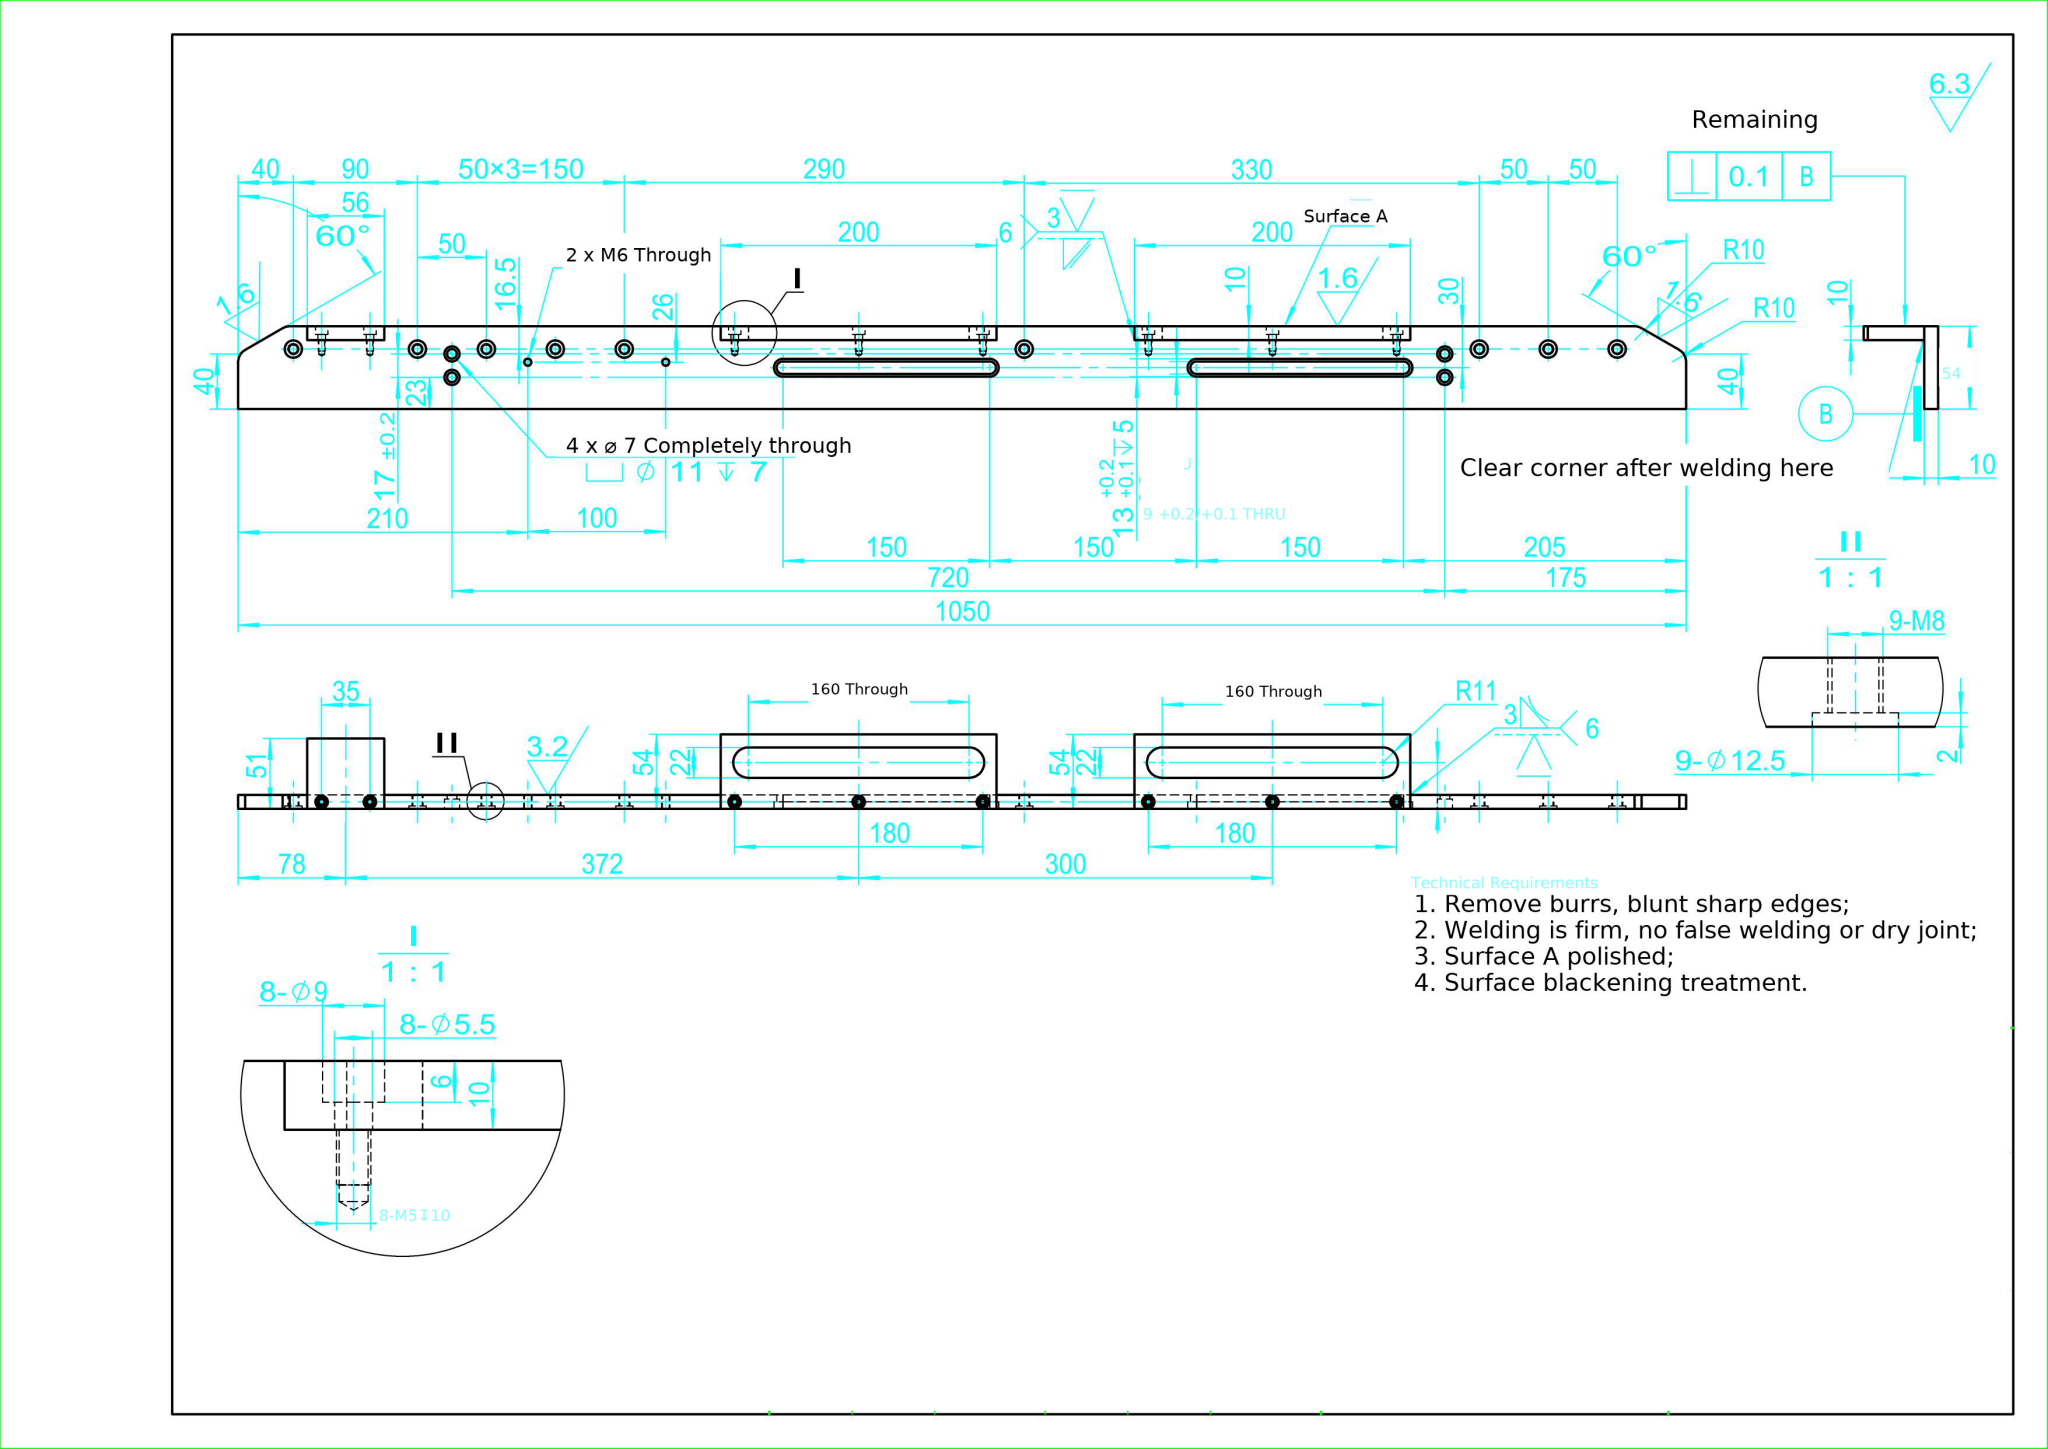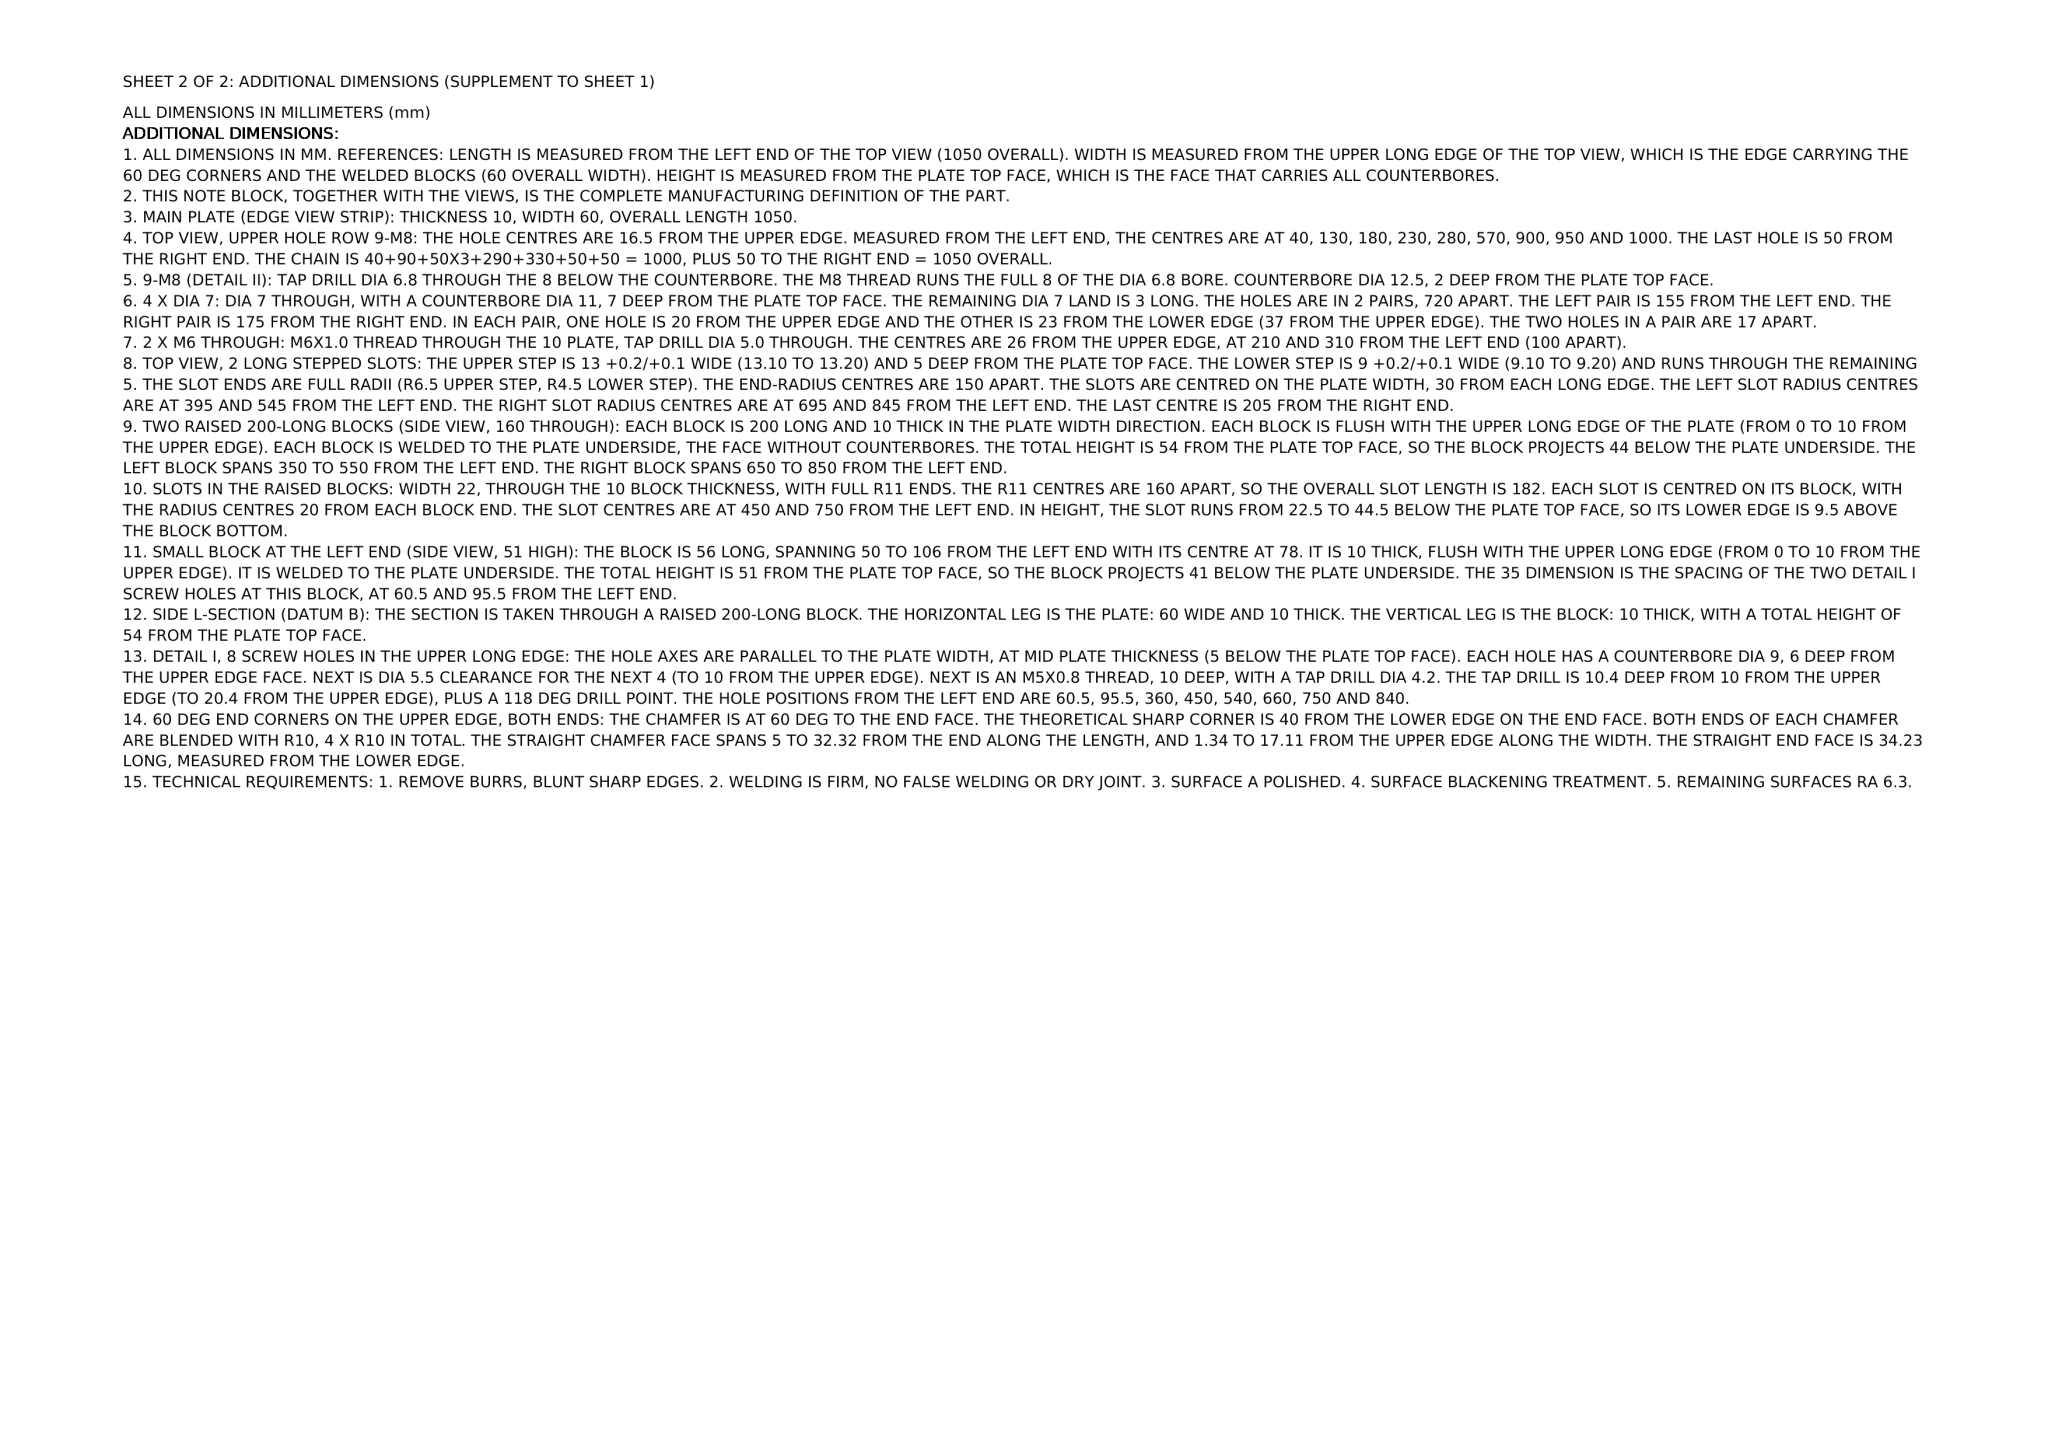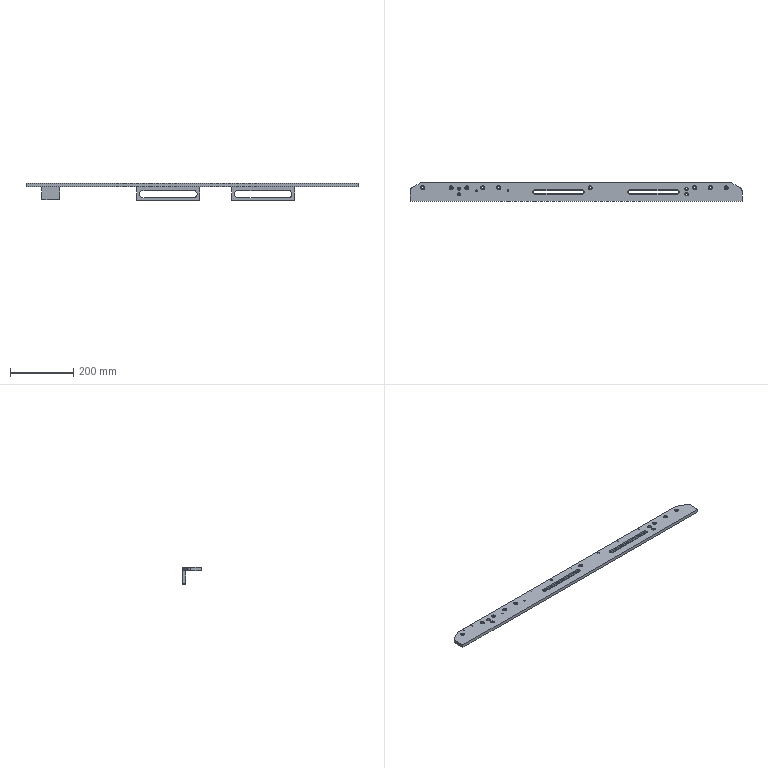Part | NX | mm | 1 solid | 205 faces | box 1050 x 60 x 54 mm | volume 695593 mm3 | cylinder 126 | plane 63 | cone 16 | commonest cylinder face diameters 9 x22 6.8 x18 12.5 x18 5.5 x16 4.2 x16 11 x8 7 x8 22 x6